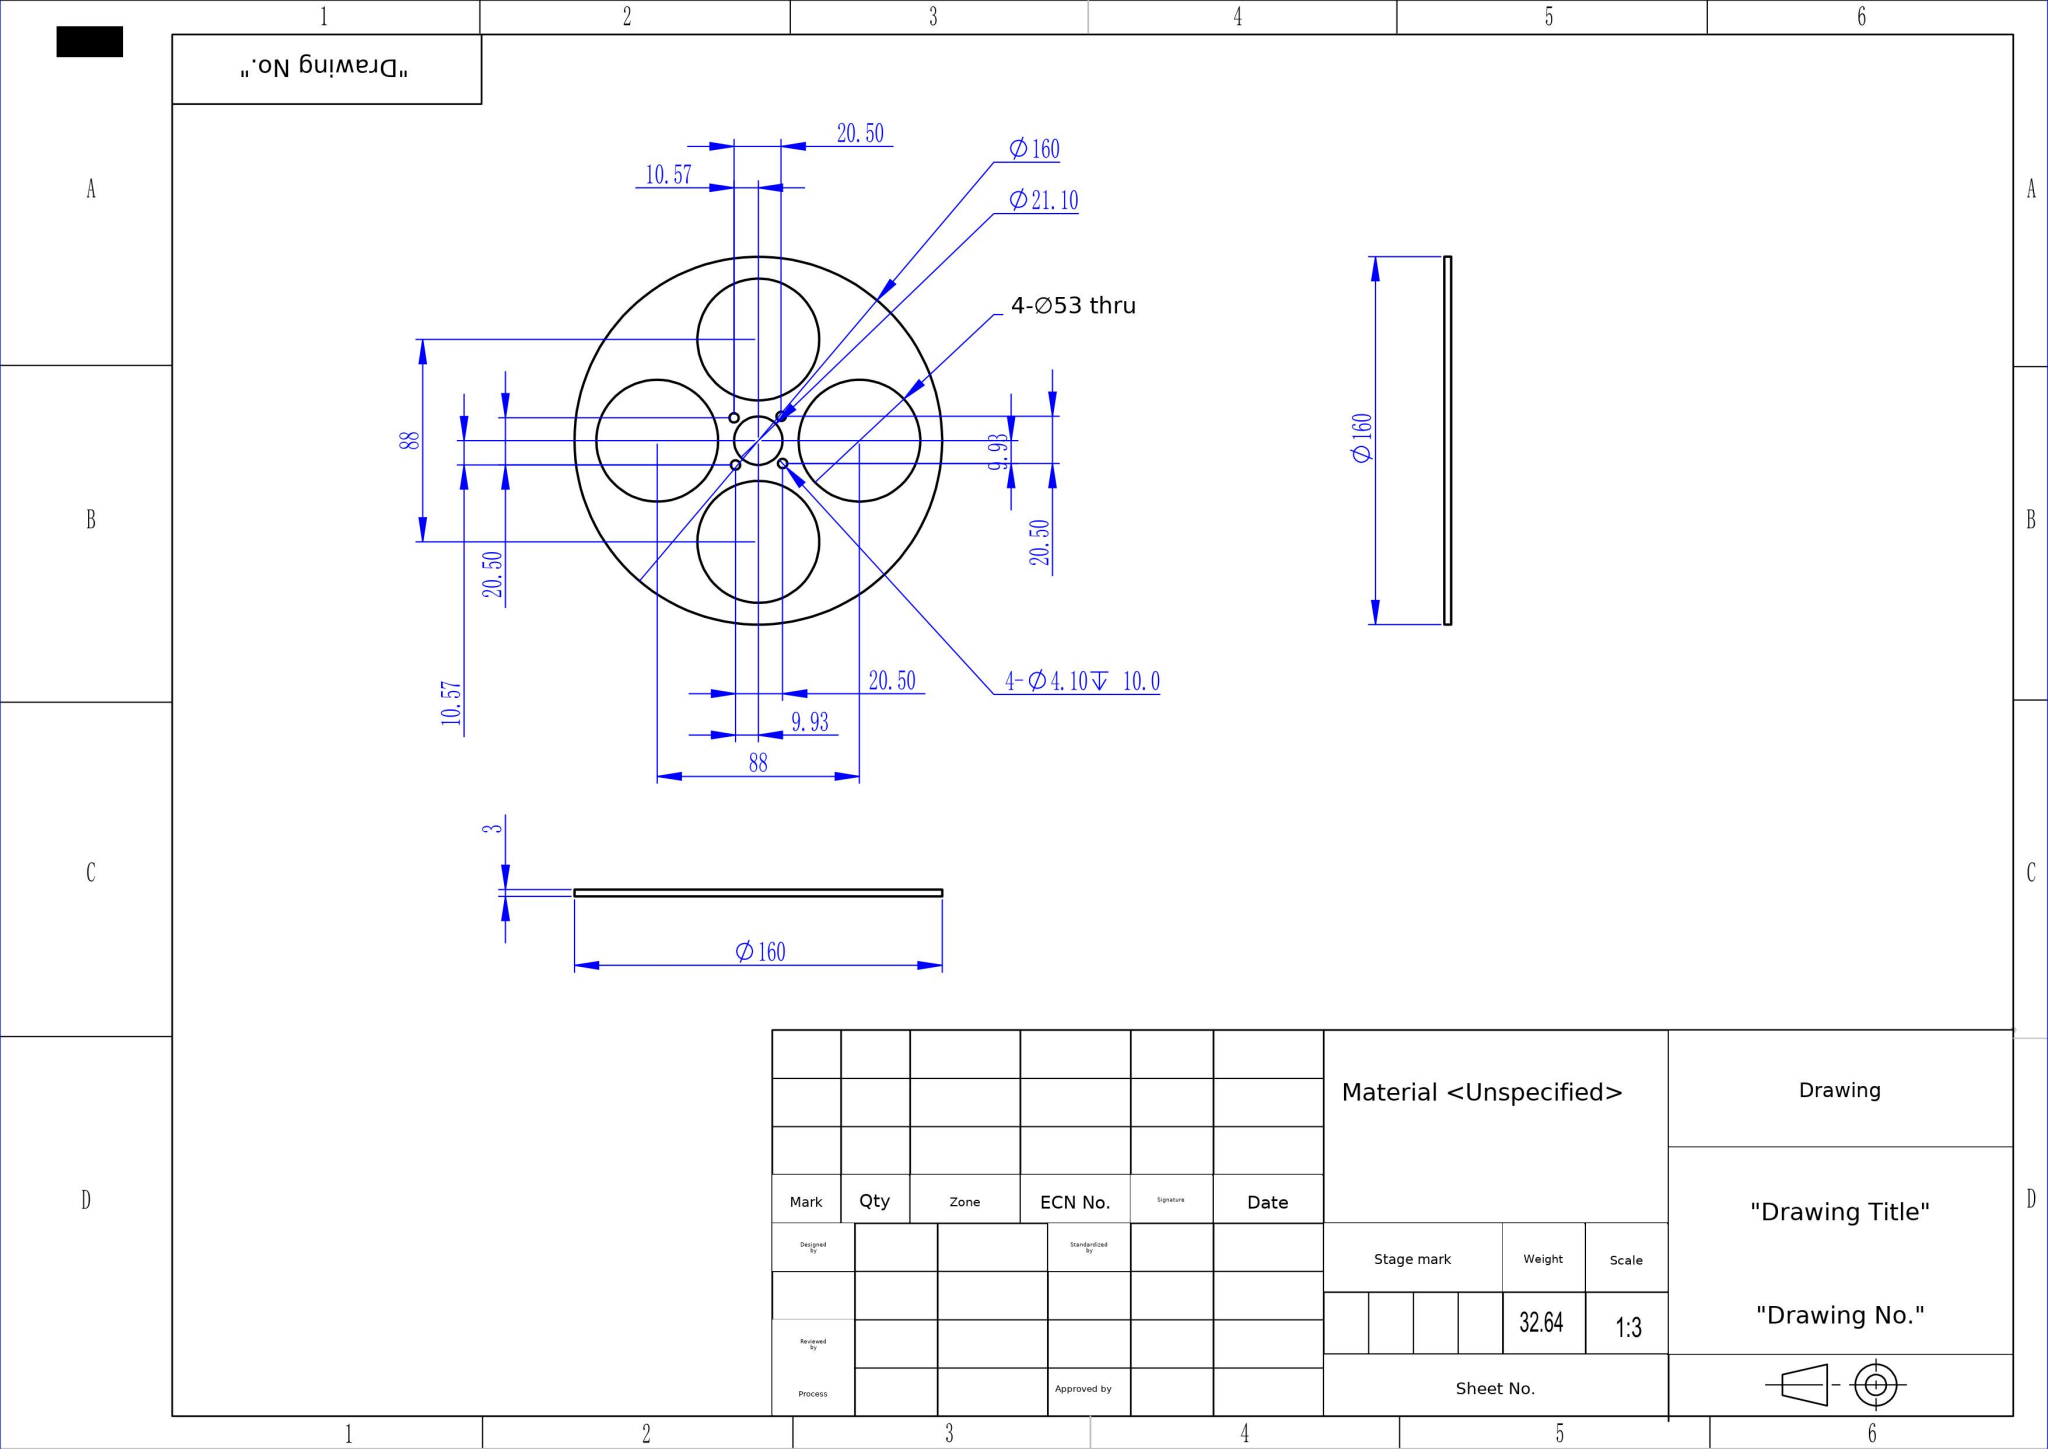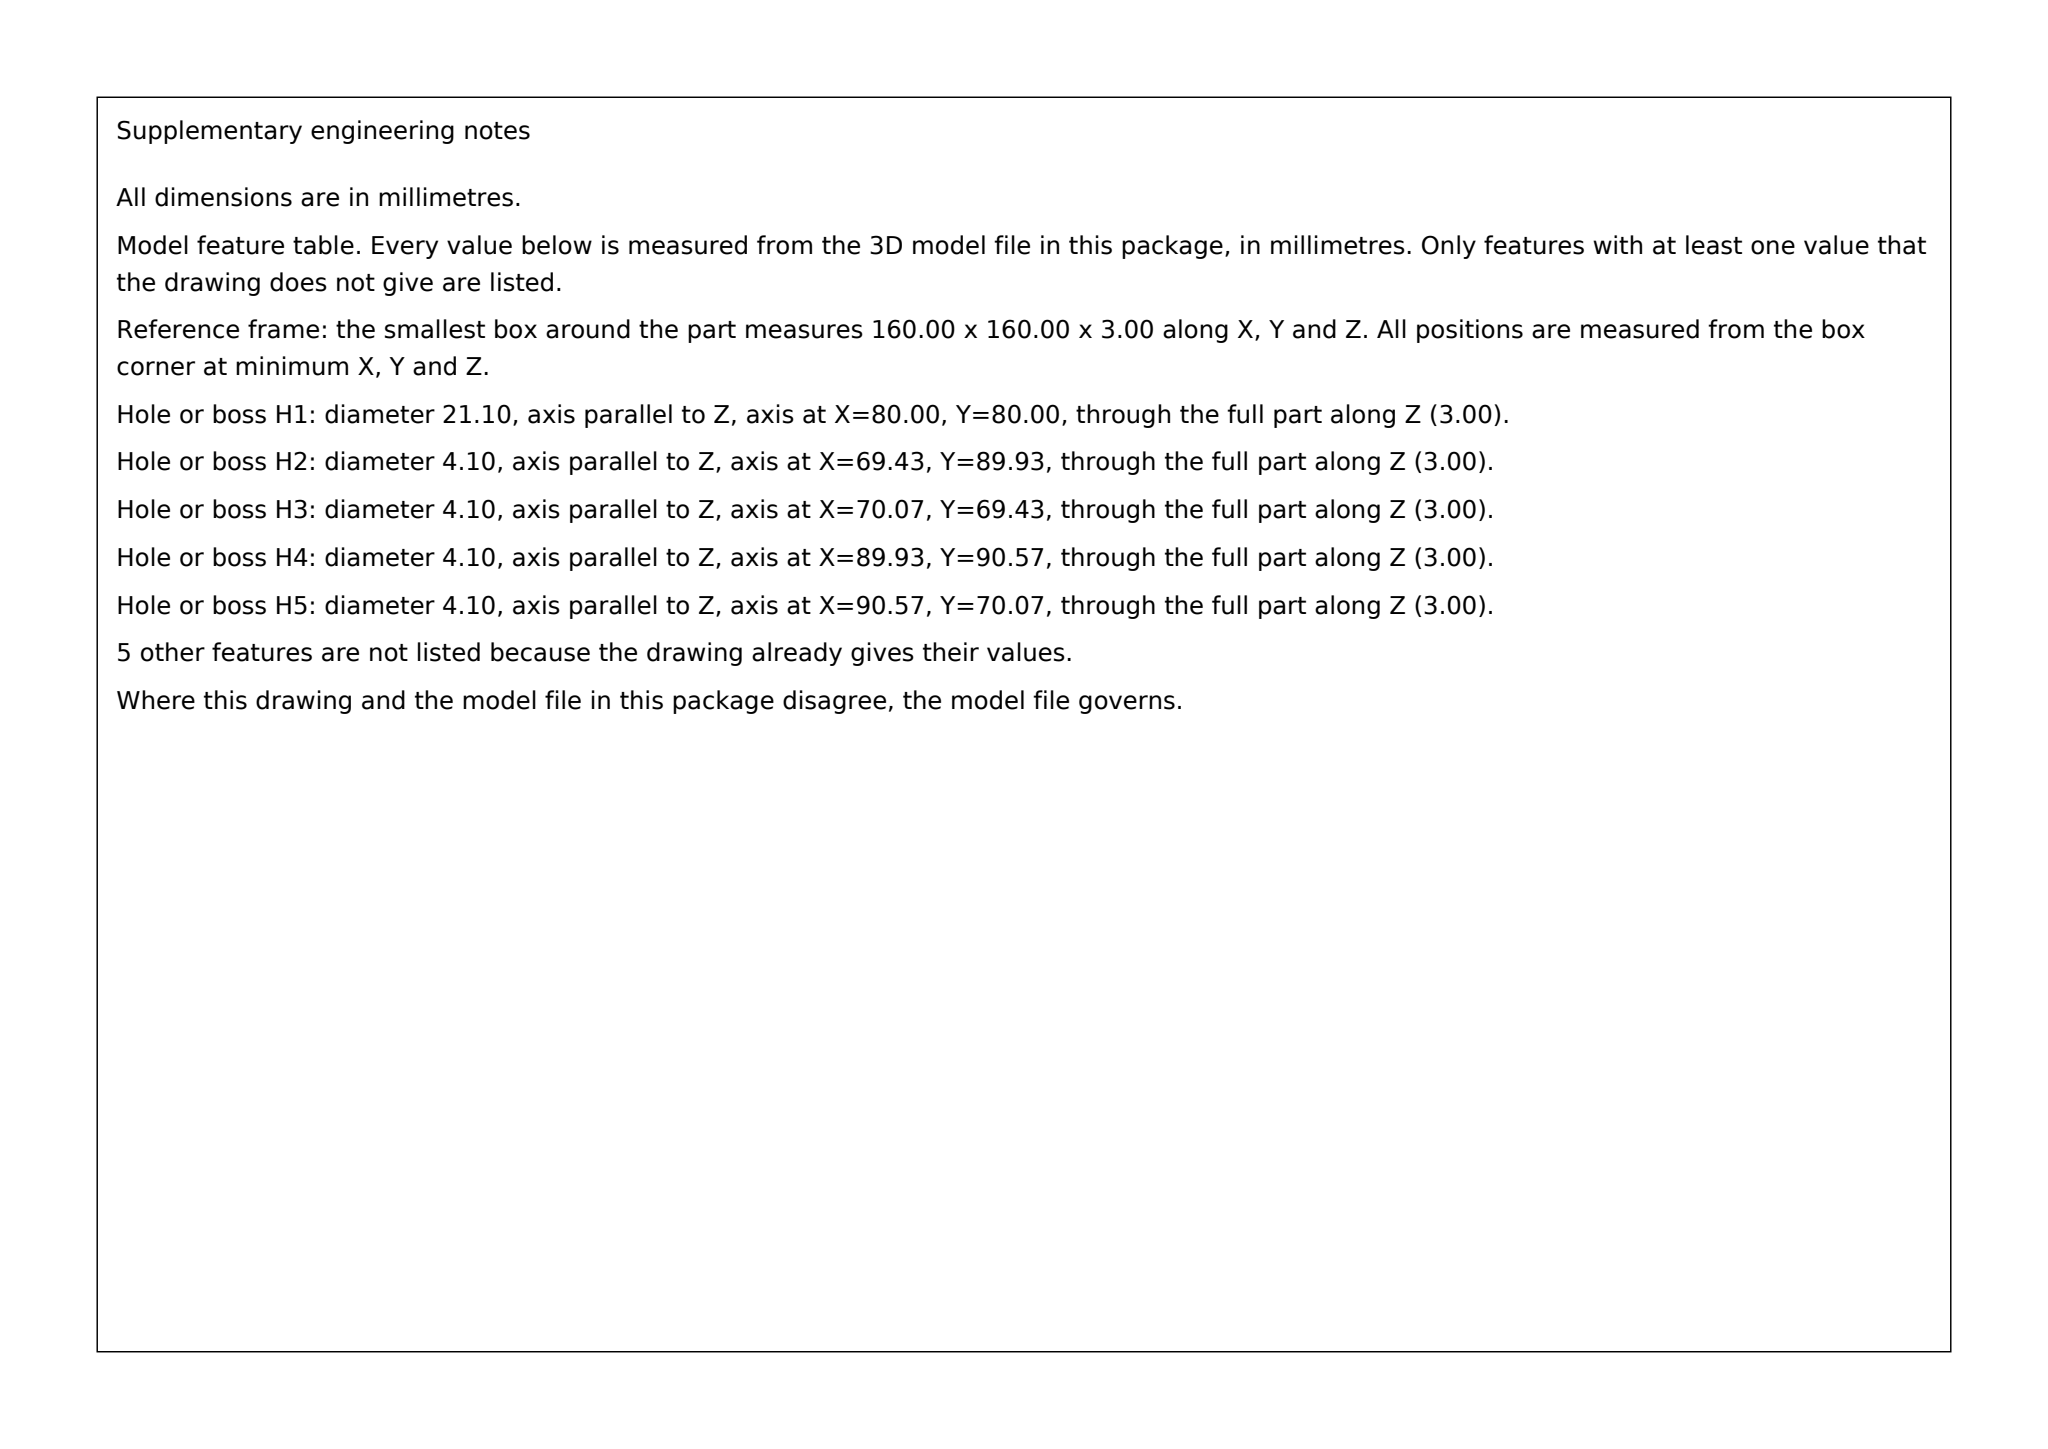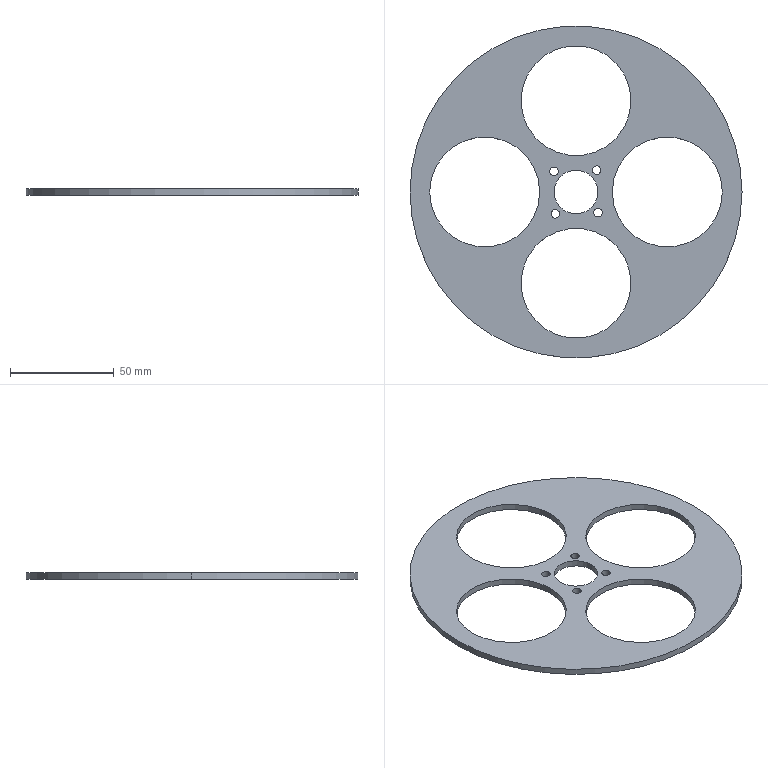Part | SolidWorks | mm | 1 solid | 22 faces | box 160 x 160 x 3 mm | volume 32637 mm3 | cylinder 20 | plane 2 | commonest cylinder face diameters 4.1 x8 53 x8 21.1 x2 160 x2
build123d program:
from build123d import *

# Parameters (mm, degrees)
SKETCH1_R           = 80
SKETCH1_R_2         = 10.55
BOSS_EXTRUDE1_DEPTH = 3
CUT_EXTRUDE1_REACH  = 115.177
SKETCH2_R           = 26.5
CIRPATTERN1_COUNT   = 4
SKETCH3_R           = 2.05
CUT_EXTRUDE2_DEPTH  = 10


with BuildPart() as part:
    # Sketch1 → Boss-Extrude1 (new body)
    with BuildSketch(Plane.XY):
        Circle(SKETCH1_R)
        Circle(SKETCH1_R_2, mode=Mode.SUBTRACT)
    extrude(amount=BOSS_EXTRUDE1_DEPTH)

    # Sketch2 → Cut-Extrude1 (cut, up to next)
    with BuildSketch(Plane.XY.offset(3), mode=Mode.PRIVATE) as cut_extrude1_sk1:
        with Locations((0, 44)):
            Circle(SKETCH2_R)
    cut_extrude1_tool1 = extrude(cut_extrude1_sk1.sketch, amount=-CUT_EXTRUDE1_REACH, mode=Mode.PRIVATE) & part.part
    cut_extrude1 = cut_extrude1_tool1.solids().sort_by_distance((0, 44, 3))[0]
    add(cut_extrude1, mode=Mode.SUBTRACT)

    # CirPattern1: Cut-Extrude1 ×4 about axis
    cirpattern1_axis = Axis((0, 0, 0), (0, 0, 1))
    for i in range(1, CIRPATTERN1_COUNT):
        add(cut_extrude1.rotate(cirpattern1_axis, i * 360 / CIRPATTERN1_COUNT), mode=Mode.SUBTRACT)

    # Sketch3 → Cut-Extrude2 (cut)
    with BuildSketch(Plane.XY.offset(3)):
        with Locations((9.929, 10.567)):
            Circle(SKETCH3_R)
        with Locations((10.567, -9.929)):
            Circle(SKETCH3_R)
        with Locations((-9.929, -10.567)):
            Circle(SKETCH3_R)
        with Locations((-10.567, 9.929)):
            Circle(SKETCH3_R)
    extrude(amount=-CUT_EXTRUDE2_DEPTH, mode=Mode.SUBTRACT)


solid = part.part
STEP:
#1=CARTESIAN_POINT('',(-12.617,9.929,0.));
#2=VERTEX_POINT('',#1);
#3=CARTESIAN_POINT('',(-8.517,9.929,0.));
#4=VERTEX_POINT('',#3);
#5=CARTESIAN_POINT('',(-10.567,9.929,0.));
#6=DIRECTION('',(0.,0.,1.));
#7=DIRECTION('',(1.,0.,0.));
#8=AXIS2_PLACEMENT_3D('',#5,#6,#7);
#9=CIRCLE('',#8,2.05);
#10=EDGE_CURVE('',#2,#4,#9,.T.);
#11=ORIENTED_EDGE('',*,*,#10,.F.);
#12=CARTESIAN_POINT('',(-12.617,9.929,3.));
#13=VERTEX_POINT('',#12);
#14=CARTESIAN_POINT('',(-12.617,9.929,-7.));
#15=DIRECTION('',(0.,0.,1.));
#16=VECTOR('',#15,1000.);
#17=LINE('',#14,#16);
#18=EDGE_CURVE('',#2,#13,#17,.T.);
#19=ORIENTED_EDGE('',*,*,#18,.T.);
#20=CARTESIAN_POINT('',(-8.517,9.929,3.));
#21=VERTEX_POINT('',#20);
#22=CARTESIAN_POINT('',(-10.567,9.929,3.));
#23=DIRECTION('',(0.,0.,1.));
#24=DIRECTION('',(1.,0.,0.));
#25=AXIS2_PLACEMENT_3D('',#22,#23,#24);
#26=CIRCLE('',#25,2.05);
#27=EDGE_CURVE('',#13,#21,#26,.T.);
#28=ORIENTED_EDGE('',*,*,#27,.T.);
#29=CARTESIAN_POINT('',(-8.517,9.929,-7.));
#30=DIRECTION('',(0.,0.,1.));
#31=VECTOR('',#30,1000.);
#32=LINE('',#29,#31);
#33=EDGE_CURVE('',#4,#21,#32,.T.);
#34=ORIENTED_EDGE('',*,*,#33,.F.);
#35=EDGE_LOOP('',(#11,#19,#28,#34));
#36=FACE_OUTER_BOUND('',#35,.T.);
#37=CARTESIAN_POINT('',(-10.567,9.929,-7.));
#38=DIRECTION('',(0.,0.,1.));
#39=DIRECTION('',(1.,0.,0.));
#40=AXIS2_PLACEMENT_3D('',#37,#38,#39);
#41=CYLINDRICAL_SURFACE('',#40,2.05);
#42=ADVANCED_FACE('',(#36),#41,.F.);
#43=CARTESIAN_POINT('',(-11.979,-10.567,0.));
#44=VERTEX_POINT('',#43);
#45=CARTESIAN_POINT('',(-7.879,-10.567,0.));
#46=VERTEX_POINT('',#45);
#47=CARTESIAN_POINT('',(-9.929,-10.567,0.));
#48=DIRECTION('',(0.,0.,1.));
#49=DIRECTION('',(1.,0.,0.));
#50=AXIS2_PLACEMENT_3D('',#47,#48,#49);
#51=CIRCLE('',#50,2.05);
#52=EDGE_CURVE('',#44,#46,#51,.T.);
#53=ORIENTED_EDGE('',*,*,#52,.F.);
#54=CARTESIAN_POINT('',(-11.979,-10.567,3.));
#55=VERTEX_POINT('',#54);
#56=CARTESIAN_POINT('',(-11.979,-10.567,-7.));
#57=DIRECTION('',(0.,0.,1.));
#58=VECTOR('',#57,1000.);
#59=LINE('',#56,#58);
#60=EDGE_CURVE('',#44,#55,#59,.T.);
#61=ORIENTED_EDGE('',*,*,#60,.T.);
#62=CARTESIAN_POINT('',(-7.879,-10.567,3.));
#63=VERTEX_POINT('',#62);
#64=CARTESIAN_POINT('',(-9.929,-10.567,3.));
#65=DIRECTION('',(0.,0.,1.));
#66=DIRECTION('',(1.,0.,0.));
#67=AXIS2_PLACEMENT_3D('',#64,#65,#66);
#68=CIRCLE('',#67,2.05);
#69=EDGE_CURVE('',#55,#63,#68,.T.);
#70=ORIENTED_EDGE('',*,*,#69,.T.);
#71=CARTESIAN_POINT('',(-7.879,-10.567,-7.));
#72=DIRECTION('',(0.,0.,1.));
#73=VECTOR('',#72,1000.);
#74=LINE('',#71,#73);
#75=EDGE_CURVE('',#46,#63,#74,.T.);
#76=ORIENTED_EDGE('',*,*,#75,.F.);
#77=EDGE_LOOP('',(#53,#61,#70,#76));
#78=FACE_OUTER_BOUND('',#77,.T.);
#79=CARTESIAN_POINT('',(-9.929,-10.567,-7.));
#80=DIRECTION('',(0.,0.,1.));
#81=DIRECTION('',(1.,0.,0.));
#82=AXIS2_PLACEMENT_3D('',#79,#80,#81);
#83=CYLINDRICAL_SURFACE('',#82,2.05);
#84=ADVANCED_FACE('',(#78),#83,.F.);
#85=CARTESIAN_POINT('',(8.517,-9.929,0.));
#86=VERTEX_POINT('',#85);
#87=CARTESIAN_POINT('',(12.617,-9.929,0.));
#88=VERTEX_POINT('',#87);
#89=CARTESIAN_POINT('',(10.567,-9.929,0.));
#90=DIRECTION('',(0.,0.,1.));
#91=DIRECTION('',(1.,0.,0.));
#92=AXIS2_PLACEMENT_3D('',#89,#90,#91);
#93=CIRCLE('',#92,2.05);
#94=EDGE_CURVE('',#86,#88,#93,.T.);
#95=ORIENTED_EDGE('',*,*,#94,.F.);
#96=CARTESIAN_POINT('',(8.517,-9.929,3.));
#97=VERTEX_POINT('',#96);
#98=CARTESIAN_POINT('',(8.517,-9.929,-7.));
#99=DIRECTION('',(0.,0.,1.));
#100=VECTOR('',#99,1000.);
#101=LINE('',#98,#100);
#102=EDGE_CURVE('',#86,#97,#101,.T.);
#103=ORIENTED_EDGE('',*,*,#102,.T.);
#104=CARTESIAN_POINT('',(12.617,-9.929,3.));
#105=VERTEX_POINT('',#104);
#106=CARTESIAN_POINT('',(10.567,-9.929,3.));
#107=DIRECTION('',(0.,0.,1.));
#108=DIRECTION('',(1.,0.,0.));
#109=AXIS2_PLACEMENT_3D('',#106,#107,#108);
#110=CIRCLE('',#109,2.05);
#111=EDGE_CURVE('',#97,#105,#110,.T.);
#112=ORIENTED_EDGE('',*,*,#111,.T.);
#113=CARTESIAN_POINT('',(12.617,-9.929,-7.));
#114=DIRECTION('',(0.,0.,1.));
#115=VECTOR('',#114,1000.);
#116=LINE('',#113,#115);
#117=EDGE_CURVE('',#88,#105,#116,.T.);
#118=ORIENTED_EDGE('',*,*,#117,.F.);
#119=EDGE_LOOP('',(#95,#103,#112,#118));
#120=FACE_OUTER_BOUND('',#119,.T.);
#121=CARTESIAN_POINT('',(10.567,-9.929,-7.));
#122=DIRECTION('',(0.,0.,1.));
#123=DIRECTION('',(1.,0.,0.));
#124=AXIS2_PLACEMENT_3D('',#121,#122,#123);
#125=CYLINDRICAL_SURFACE('',#124,2.05);
#126=ADVANCED_FACE('',(#120),#125,.F.);
#127=CARTESIAN_POINT('',(7.879,10.567,0.));
#128=VERTEX_POINT('',#127);
#129=CARTESIAN_POINT('',(11.979,10.567,0.));
#130=VERTEX_POINT('',#129);
#131=CARTESIAN_POINT('',(9.929,10.567,0.));
#132=DIRECTION('',(0.,0.,1.));
#133=DIRECTION('',(1.,0.,0.));
#134=AXIS2_PLACEMENT_3D('',#131,#132,#133);
#135=CIRCLE('',#134,2.05);
#136=EDGE_CURVE('',#128,#130,#135,.T.);
#137=ORIENTED_EDGE('',*,*,#136,.F.);
#138=CARTESIAN_POINT('',(7.879,10.567,3.));
#139=VERTEX_POINT('',#138);
#140=CARTESIAN_POINT('',(7.879,10.567,-7.));
#141=DIRECTION('',(0.,0.,1.));
#142=VECTOR('',#141,1000.);
#143=LINE('',#140,#142);
#144=EDGE_CURVE('',#128,#139,#143,.T.);
#145=ORIENTED_EDGE('',*,*,#144,.T.);
#146=CARTESIAN_POINT('',(11.979,10.567,3.));
#147=VERTEX_POINT('',#146);
#148=CARTESIAN_POINT('',(9.929,10.567,3.));
#149=DIRECTION('',(0.,0.,1.));
#150=DIRECTION('',(1.,0.,0.));
#151=AXIS2_PLACEMENT_3D('',#148,#149,#150);
#152=CIRCLE('',#151,2.05);
#153=EDGE_CURVE('',#139,#147,#152,.T.);
#154=ORIENTED_EDGE('',*,*,#153,.T.);
#155=CARTESIAN_POINT('',(11.979,10.567,-7.));
#156=DIRECTION('',(0.,0.,1.));
#157=VECTOR('',#156,1000.);
#158=LINE('',#155,#157);
#159=EDGE_CURVE('',#130,#147,#158,.T.);
#160=ORIENTED_EDGE('',*,*,#159,.F.);
#161=EDGE_LOOP('',(#137,#145,#154,#160));
#162=FACE_OUTER_BOUND('',#161,.T.);
#163=CARTESIAN_POINT('',(9.929,10.567,-7.));
#164=DIRECTION('',(0.,0.,1.));
#165=DIRECTION('',(1.,0.,0.));
#166=AXIS2_PLACEMENT_3D('',#163,#164,#165);
#167=CYLINDRICAL_SURFACE('',#166,2.05);
#168=ADVANCED_FACE('',(#162),#167,.F.);
#169=CARTESIAN_POINT('',(26.5,-44.,0.));
#170=VERTEX_POINT('',#169);
#171=CARTESIAN_POINT('',(-26.5,-44.,0.));
#172=VERTEX_POINT('',#171);
#173=CARTESIAN_POINT('',(0.,-44.,0.));
#174=DIRECTION('',(0.,0.,-1.));
#175=DIRECTION('',(1.,0.,0.));
#176=AXIS2_PLACEMENT_3D('',#173,#174,#175);
#177=CIRCLE('',#176,26.5);
#178=EDGE_CURVE('',#170,#172,#177,.T.);
#179=ORIENTED_EDGE('',*,*,#178,.T.);
#180=CARTESIAN_POINT('',(-26.5,-44.,3.));
#181=VERTEX_POINT('',#180);
#182=CARTESIAN_POINT('',(-26.5,-44.,-0.001));
#183=DIRECTION('',(0.,0.,1.));
#184=VECTOR('',#183,1000.);
#185=LINE('',#182,#184);
#186=EDGE_CURVE('',#172,#181,#185,.T.);
#187=ORIENTED_EDGE('',*,*,#186,.T.);
#188=CARTESIAN_POINT('',(26.5,-44.,3.));
#189=VERTEX_POINT('',#188);
#190=CARTESIAN_POINT('',(0.,-44.,3.));
#191=DIRECTION('',(0.,0.,1.));
#192=DIRECTION('',(-1.,0.,0.));
#193=AXIS2_PLACEMENT_3D('',#190,#191,#192);
#194=CIRCLE('',#193,26.5);
#195=EDGE_CURVE('',#181,#189,#194,.T.);
#196=ORIENTED_EDGE('',*,*,#195,.T.);
#197=CARTESIAN_POINT('',(26.5,-44.,-0.001));
#198=DIRECTION('',(0.,0.,1.));
#199=VECTOR('',#198,1000.);
#200=LINE('',#197,#199);
#201=EDGE_CURVE('',#170,#189,#200,.T.);
#202=ORIENTED_EDGE('',*,*,#201,.F.);
#203=EDGE_LOOP('',(#179,#187,#196,#202));
#204=FACE_OUTER_BOUND('',#203,.T.);
#205=CARTESIAN_POINT('',(0.,-44.,-0.001));
#206=DIRECTION('',(0.,0.,1.));
#207=DIRECTION('',(1.,0.,0.));
#208=AXIS2_PLACEMENT_3D('',#205,#206,#207);
#209=CYLINDRICAL_SURFACE('',#208,26.5);
#210=ADVANCED_FACE('',(#204),#209,.F.);
#211=CARTESIAN_POINT('',(-17.5,0.,0.));
#212=VERTEX_POINT('',#211);
#213=CARTESIAN_POINT('',(-70.5,0.,0.));
#214=VERTEX_POINT('',#213);
#215=CARTESIAN_POINT('',(-44.,0.,0.));
#216=DIRECTION('',(0.,0.,-1.));
#217=DIRECTION('',(1.,0.,0.));
#218=AXIS2_PLACEMENT_3D('',#215,#216,#217);
#219=CIRCLE('',#218,26.5);
#220=EDGE_CURVE('',#212,#214,#219,.T.);
#221=ORIENTED_EDGE('',*,*,#220,.T.);
#222=CARTESIAN_POINT('',(-70.5,0.,3.));
#223=VERTEX_POINT('',#222);
#224=CARTESIAN_POINT('',(-70.5,0.,-0.001));
#225=DIRECTION('',(0.,0.,1.));
#226=VECTOR('',#225,1000.);
#227=LINE('',#224,#226);
#228=EDGE_CURVE('',#214,#223,#227,.T.);
#229=ORIENTED_EDGE('',*,*,#228,.T.);
#230=CARTESIAN_POINT('',(-17.5,0.,3.));
#231=VERTEX_POINT('',#230);
#232=CARTESIAN_POINT('',(-44.,0.,3.));
#233=DIRECTION('',(0.,0.,1.));
#234=DIRECTION('',(0.,1.,0.));
#235=AXIS2_PLACEMENT_3D('',#232,#233,#234);
#236=CIRCLE('',#235,26.5);
#237=EDGE_CURVE('',#223,#231,#236,.T.);
#238=ORIENTED_EDGE('',*,*,#237,.T.);
#239=CARTESIAN_POINT('',(-17.5,0.,-0.001));
#240=DIRECTION('',(0.,0.,1.));
#241=VECTOR('',#240,1000.);
#242=LINE('',#239,#241);
#243=EDGE_CURVE('',#212,#231,#242,.T.);
#244=ORIENTED_EDGE('',*,*,#243,.F.);
#245=EDGE_LOOP('',(#221,#229,#238,#244));
#246=FACE_OUTER_BOUND('',#245,.T.);
#247=CARTESIAN_POINT('',(-44.,0.,-0.001));
#248=DIRECTION('',(0.,0.,1.));
#249=DIRECTION('',(1.,0.,0.));
#250=AXIS2_PLACEMENT_3D('',#247,#248,#249);
#251=CYLINDRICAL_SURFACE('',#250,26.5);
#252=ADVANCED_FACE('',(#246),#251,.F.);
#253=CARTESIAN_POINT('',(70.5,-0.,0.));
#254=VERTEX_POINT('',#253);
#255=CARTESIAN_POINT('',(17.5,-0.,0.));
#256=VERTEX_POINT('',#255);
#257=CARTESIAN_POINT('',(44.,-0.,0.));
#258=DIRECTION('',(0.,0.,-1.));
#259=DIRECTION('',(1.,0.,0.));
#260=AXIS2_PLACEMENT_3D('',#257,#258,#259);
#261=CIRCLE('',#260,26.5);
#262=EDGE_CURVE('',#254,#256,#261,.T.);
#263=ORIENTED_EDGE('',*,*,#262,.T.);
#264=CARTESIAN_POINT('',(17.5,-0.,3.));
#265=VERTEX_POINT('',#264);
#266=CARTESIAN_POINT('',(17.5,-0.,-0.001));
#267=DIRECTION('',(0.,0.,1.));
#268=VECTOR('',#267,1000.);
#269=LINE('',#266,#268);
#270=EDGE_CURVE('',#256,#265,#269,.T.);
#271=ORIENTED_EDGE('',*,*,#270,.T.);
#272=CARTESIAN_POINT('',(70.5,-0.,3.));
#273=VERTEX_POINT('',#272);
#274=CARTESIAN_POINT('',(44.,-0.,3.));
#275=DIRECTION('',(0.,0.,1.));
#276=DIRECTION('',(-0.,-1.,0.));
#277=AXIS2_PLACEMENT_3D('',#274,#275,#276);
#278=CIRCLE('',#277,26.5);
#279=EDGE_CURVE('',#265,#273,#278,.T.);
#280=ORIENTED_EDGE('',*,*,#279,.T.);
#281=CARTESIAN_POINT('',(70.5,-0.,-0.001));
#282=DIRECTION('',(0.,0.,1.));
#283=VECTOR('',#282,1000.);
#284=LINE('',#281,#283);
#285=EDGE_CURVE('',#254,#273,#284,.T.);
#286=ORIENTED_EDGE('',*,*,#285,.F.);
#287=EDGE_LOOP('',(#263,#271,#280,#286));
#288=FACE_OUTER_BOUND('',#287,.T.);
#289=CARTESIAN_POINT('',(44.,-0.,-0.001));
#290=DIRECTION('',(0.,0.,1.));
#291=DIRECTION('',(1.,0.,0.));
#292=AXIS2_PLACEMENT_3D('',#289,#290,#291);
#293=CYLINDRICAL_SURFACE('',#292,26.5);
#294=ADVANCED_FACE('',(#288),#293,.F.);
#295=CARTESIAN_POINT('',(26.5,44.,0.));
#296=VERTEX_POINT('',#295);
#297=CARTESIAN_POINT('',(-26.5,44.,0.));
#298=VERTEX_POINT('',#297);
#299=CARTESIAN_POINT('',(0.,44.,0.));
#300=DIRECTION('',(0.,0.,-1.));
#301=DIRECTION('',(1.,0.,0.));
#302=AXIS2_PLACEMENT_3D('',#299,#300,#301);
#303=CIRCLE('',#302,26.5);
#304=EDGE_CURVE('',#296,#298,#303,.T.);
#305=ORIENTED_EDGE('',*,*,#304,.T.);
#306=CARTESIAN_POINT('',(-26.5,44.,3.));
#307=VERTEX_POINT('',#306);
#308=CARTESIAN_POINT('',(-26.5,44.,-0.001));
#309=DIRECTION('',(0.,0.,1.));
#310=VECTOR('',#309,1000.);
#311=LINE('',#308,#310);
#312=EDGE_CURVE('',#298,#307,#311,.T.);
#313=ORIENTED_EDGE('',*,*,#312,.T.);
#314=CARTESIAN_POINT('',(26.5,44.,3.));
#315=VERTEX_POINT('',#314);
#316=CARTESIAN_POINT('',(0.,44.,3.));
#317=DIRECTION('',(0.,0.,1.));
#318=DIRECTION('',(1.,0.,0.));
#319=AXIS2_PLACEMENT_3D('',#316,#317,#318);
#320=CIRCLE('',#319,26.5);
#321=EDGE_CURVE('',#307,#315,#320,.T.);
#322=ORIENTED_EDGE('',*,*,#321,.T.);
#323=CARTESIAN_POINT('',(26.5,44.,-0.001));
#324=DIRECTION('',(0.,0.,1.));
#325=VECTOR('',#324,1000.);
#326=LINE('',#323,#325);
#327=EDGE_CURVE('',#296,#315,#326,.T.);
#328=ORIENTED_EDGE('',*,*,#327,.F.);
#329=EDGE_LOOP('',(#305,#313,#322,#328));
#330=FACE_OUTER_BOUND('',#329,.T.);
#331=CARTESIAN_POINT('',(0.,44.,-0.001));
#332=DIRECTION('',(0.,0.,1.));
#333=DIRECTION('',(1.,0.,0.));
#334=AXIS2_PLACEMENT_3D('',#331,#332,#333);
#335=CYLINDRICAL_SURFACE('',#334,26.5);
#336=ADVANCED_FACE('',(#330),#335,.F.);
#337=CARTESIAN_POINT('',(-10.55,0.,3.));
#338=VERTEX_POINT('',#337);
#339=CARTESIAN_POINT('',(10.55,0.,3.));
#340=VERTEX_POINT('',#339);
#341=CARTESIAN_POINT('',(0.,0.,3.));
#342=DIRECTION('',(0.,0.,1.));
#343=DIRECTION('',(1.,0.,0.));
#344=AXIS2_PLACEMENT_3D('',#341,#342,#343);
#345=CIRCLE('',#344,10.55);
#346=EDGE_CURVE('',#338,#340,#345,.T.);
#347=ORIENTED_EDGE('',*,*,#346,.T.);
#348=CARTESIAN_POINT('',(10.55,0.,0.));
#349=VERTEX_POINT('',#348);
#350=CARTESIAN_POINT('',(10.55,0.,3.));
#351=DIRECTION('',(0.,0.,-1.));
#352=VECTOR('',#351,1000.);
#353=LINE('',#350,#352);
#354=EDGE_CURVE('',#340,#349,#353,.T.);
#355=ORIENTED_EDGE('',*,*,#354,.T.);
#356=CARTESIAN_POINT('',(-10.55,0.,0.));
#357=VERTEX_POINT('',#356);
#358=CARTESIAN_POINT('',(0.,0.,0.));
#359=DIRECTION('',(0.,0.,1.));
#360=DIRECTION('',(1.,0.,0.));
#361=AXIS2_PLACEMENT_3D('',#358,#359,#360);
#362=CIRCLE('',#361,10.55);
#363=EDGE_CURVE('',#357,#349,#362,.T.);
#364=ORIENTED_EDGE('',*,*,#363,.F.);
#365=CARTESIAN_POINT('',(-10.55,0.,3.));
#366=DIRECTION('',(0.,0.,-1.));
#367=VECTOR('',#366,1000.);
#368=LINE('',#365,#367);
#369=EDGE_CURVE('',#338,#357,#368,.T.);
#370=ORIENTED_EDGE('',*,*,#369,.F.);
#371=EDGE_LOOP('',(#347,#355,#364,#370));
#372=FACE_OUTER_BOUND('',#371,.T.);
#373=CARTESIAN_POINT('',(0.,0.,3.));
#374=DIRECTION('',(0.,0.,-1.));
#375=DIRECTION('',(-1.,0.,0.));
#376=AXIS2_PLACEMENT_3D('',#373,#374,#375);
#377=CYLINDRICAL_SURFACE('',#376,10.55);
#378=ADVANCED_FACE('',(#372),#377,.F.);
#379=CARTESIAN_POINT('',(80.,0.,3.));
#380=VERTEX_POINT('',#379);
#381=CARTESIAN_POINT('',(-80.,0.,3.));
#382=VERTEX_POINT('',#381);
#383=CARTESIAN_POINT('',(0.,0.,3.));
#384=DIRECTION('',(0.,0.,1.));
#385=DIRECTION('',(1.,0.,0.));
#386=AXIS2_PLACEMENT_3D('',#383,#384,#385);
#387=CIRCLE('',#386,80.);
#388=EDGE_CURVE('',#380,#382,#387,.T.);
#389=ORIENTED_EDGE('',*,*,#388,.F.);
#390=CARTESIAN_POINT('',(80.,0.,0.));
#391=VERTEX_POINT('',#390);
#392=CARTESIAN_POINT('',(80.,0.,3.));
#393=DIRECTION('',(0.,0.,-1.));
#394=VECTOR('',#393,1000.);
#395=LINE('',#392,#394);
#396=EDGE_CURVE('',#380,#391,#395,.T.);
#397=ORIENTED_EDGE('',*,*,#396,.T.);
#398=CARTESIAN_POINT('',(-80.,0.,0.));
#399=VERTEX_POINT('',#398);
#400=CARTESIAN_POINT('',(0.,0.,0.));
#401=DIRECTION('',(0.,0.,1.));
#402=DIRECTION('',(1.,0.,0.));
#403=AXIS2_PLACEMENT_3D('',#400,#401,#402);
#404=CIRCLE('',#403,80.);
#405=EDGE_CURVE('',#391,#399,#404,.T.);
#406=ORIENTED_EDGE('',*,*,#405,.T.);
#407=CARTESIAN_POINT('',(-80.,0.,3.));
#408=DIRECTION('',(0.,0.,-1.));
#409=VECTOR('',#408,1000.);
#410=LINE('',#407,#409);
#411=EDGE_CURVE('',#382,#399,#410,.T.);
#412=ORIENTED_EDGE('',*,*,#411,.F.);
#413=EDGE_LOOP('',(#389,#397,#406,#412));
#414=FACE_OUTER_BOUND('',#413,.T.);
#415=CARTESIAN_POINT('',(0.,0.,3.));
#416=DIRECTION('',(0.,0.,-1.));
#417=DIRECTION('',(-1.,0.,0.));
#418=AXIS2_PLACEMENT_3D('',#415,#416,#417);
#419=CYLINDRICAL_SURFACE('',#418,80.);
#420=ADVANCED_FACE('',(#414),#419,.T.);
#421=CARTESIAN_POINT('',(-10.567,9.929,3.));
#422=DIRECTION('',(0.,0.,1.));
#423=DIRECTION('',(1.,0.,0.));
#424=AXIS2_PLACEMENT_3D('',#421,#422,#423);
#425=CIRCLE('',#424,2.05);
#426=EDGE_CURVE('',#21,#13,#425,.T.);
#427=ORIENTED_EDGE('',*,*,#426,.F.);
#428=ORIENTED_EDGE('',*,*,#27,.F.);
#429=EDGE_LOOP('',(#427,#428));
#430=FACE_BOUND('',#429,.T.);
#431=CARTESIAN_POINT('',(-9.929,-10.567,3.));
#432=DIRECTION('',(0.,0.,1.));
#433=DIRECTION('',(1.,0.,0.));
#434=AXIS2_PLACEMENT_3D('',#431,#432,#433);
#435=CIRCLE('',#434,2.05);
#436=EDGE_CURVE('',#63,#55,#435,.T.);
#437=ORIENTED_EDGE('',*,*,#436,.F.);
#438=ORIENTED_EDGE('',*,*,#69,.F.);
#439=EDGE_LOOP('',(#437,#438));
#440=FACE_BOUND('',#439,.T.);
#441=CARTESIAN_POINT('',(10.567,-9.929,3.));
#442=DIRECTION('',(0.,0.,1.));
#443=DIRECTION('',(1.,0.,0.));
#444=AXIS2_PLACEMENT_3D('',#441,#442,#443);
#445=CIRCLE('',#444,2.05);
#446=EDGE_CURVE('',#105,#97,#445,.T.);
#447=ORIENTED_EDGE('',*,*,#446,.F.);
#448=ORIENTED_EDGE('',*,*,#111,.F.);
#449=EDGE_LOOP('',(#447,#448));
#450=FACE_BOUND('',#449,.T.);
#451=CARTESIAN_POINT('',(9.929,10.567,3.));
#452=DIRECTION('',(0.,0.,1.));
#453=DIRECTION('',(1.,0.,0.));
#454=AXIS2_PLACEMENT_3D('',#451,#452,#453);
#455=CIRCLE('',#454,2.05);
#456=EDGE_CURVE('',#147,#139,#455,.T.);
#457=ORIENTED_EDGE('',*,*,#456,.F.);
#458=ORIENTED_EDGE('',*,*,#153,.F.);
#459=EDGE_LOOP('',(#457,#458));
#460=FACE_BOUND('',#459,.T.);
#461=CARTESIAN_POINT('',(0.,-44.,3.));
#462=DIRECTION('',(0.,0.,1.));
#463=DIRECTION('',(-1.,0.,0.));
#464=AXIS2_PLACEMENT_3D('',#461,#462,#463);
#465=CIRCLE('',#464,26.5);
#466=EDGE_CURVE('',#189,#181,#465,.T.);
#467=ORIENTED_EDGE('',*,*,#466,.F.);
#468=ORIENTED_EDGE('',*,*,#195,.F.);
#469=EDGE_LOOP('',(#467,#468));
#470=FACE_BOUND('',#469,.T.);
#471=CARTESIAN_POINT('',(-44.,0.,3.));
#472=DIRECTION('',(0.,0.,1.));
#473=DIRECTION('',(0.,1.,0.));
#474=AXIS2_PLACEMENT_3D('',#471,#472,#473);
#475=CIRCLE('',#474,26.5);
#476=EDGE_CURVE('',#231,#223,#475,.T.);
#477=ORIENTED_EDGE('',*,*,#476,.F.);
#478=ORIENTED_EDGE('',*,*,#237,.F.);
#479=EDGE_LOOP('',(#477,#478));
#480=FACE_BOUND('',#479,.T.);
#481=CARTESIAN_POINT('',(44.,-0.,3.));
#482=DIRECTION('',(0.,0.,1.));
#483=DIRECTION('',(-0.,-1.,0.));
#484=AXIS2_PLACEMENT_3D('',#481,#482,#483);
#485=CIRCLE('',#484,26.5);
#486=EDGE_CURVE('',#273,#265,#485,.T.);
#487=ORIENTED_EDGE('',*,*,#486,.F.);
#488=ORIENTED_EDGE('',*,*,#279,.F.);
#489=EDGE_LOOP('',(#487,#488));
#490=FACE_BOUND('',#489,.T.);
#491=CARTESIAN_POINT('',(0.,44.,3.));
#492=DIRECTION('',(0.,0.,1.));
#493=DIRECTION('',(1.,0.,0.));
#494=AXIS2_PLACEMENT_3D('',#491,#492,#493);
#495=CIRCLE('',#494,26.5);
#496=EDGE_CURVE('',#315,#307,#495,.T.);
#497=ORIENTED_EDGE('',*,*,#496,.F.);
#498=ORIENTED_EDGE('',*,*,#321,.F.);
#499=EDGE_LOOP('',(#497,#498));
#500=FACE_BOUND('',#499,.T.);
#501=CARTESIAN_POINT('',(0.,0.,3.));
#502=DIRECTION('',(0.,0.,1.));
#503=DIRECTION('',(1.,0.,0.));
#504=AXIS2_PLACEMENT_3D('',#501,#502,#503);
#505=CIRCLE('',#504,80.);
#506=EDGE_CURVE('',#382,#380,#505,.T.);
#507=ORIENTED_EDGE('',*,*,#506,.T.);
#508=ORIENTED_EDGE('',*,*,#388,.T.);
#509=EDGE_LOOP('',(#507,#508));
#510=FACE_OUTER_BOUND('',#509,.T.);
#511=ORIENTED_EDGE('',*,*,#346,.F.);
#512=CARTESIAN_POINT('',(0.,0.,3.));
#513=DIRECTION('',(0.,0.,1.));
#514=DIRECTION('',(1.,0.,0.));
#515=AXIS2_PLACEMENT_3D('',#512,#513,#514);
#516=CIRCLE('',#515,10.55);
#517=EDGE_CURVE('',#340,#338,#516,.T.);
#518=ORIENTED_EDGE('',*,*,#517,.F.);
#519=EDGE_LOOP('',(#511,#518));
#520=FACE_BOUND('',#519,.T.);
#521=CARTESIAN_POINT('',(0.,0.,3.));
#522=DIRECTION('',(0.,0.,1.));
#523=DIRECTION('',(1.,0.,0.));
#524=AXIS2_PLACEMENT_3D('',#521,#522,#523);
#525=PLANE('',#524);
#526=ADVANCED_FACE('',(#430,#440,#450,#460,#470,#480,#490,#500,#510,#520),#525,.T.);
#527=CARTESIAN_POINT('',(-10.567,9.929,0.));
#528=DIRECTION('',(0.,0.,1.));
#529=DIRECTION('',(1.,0.,0.));
#530=AXIS2_PLACEMENT_3D('',#527,#528,#529);
#531=CIRCLE('',#530,2.05);
#532=EDGE_CURVE('',#4,#2,#531,.T.);
#533=ORIENTED_EDGE('',*,*,#532,.T.);
#534=ORIENTED_EDGE('',*,*,#10,.T.);
#535=EDGE_LOOP('',(#533,#534));
#536=FACE_BOUND('',#535,.T.);
#537=CARTESIAN_POINT('',(-9.929,-10.567,0.));
#538=DIRECTION('',(0.,0.,1.));
#539=DIRECTION('',(1.,0.,0.));
#540=AXIS2_PLACEMENT_3D('',#537,#538,#539);
#541=CIRCLE('',#540,2.05);
#542=EDGE_CURVE('',#46,#44,#541,.T.);
#543=ORIENTED_EDGE('',*,*,#542,.T.);
#544=ORIENTED_EDGE('',*,*,#52,.T.);
#545=EDGE_LOOP('',(#543,#544));
#546=FACE_BOUND('',#545,.T.);
#547=CARTESIAN_POINT('',(10.567,-9.929,0.));
#548=DIRECTION('',(0.,0.,1.));
#549=DIRECTION('',(1.,0.,0.));
#550=AXIS2_PLACEMENT_3D('',#547,#548,#549);
#551=CIRCLE('',#550,2.05);
#552=EDGE_CURVE('',#88,#86,#551,.T.);
#553=ORIENTED_EDGE('',*,*,#552,.T.);
#554=ORIENTED_EDGE('',*,*,#94,.T.);
#555=EDGE_LOOP('',(#553,#554));
#556=FACE_BOUND('',#555,.T.);
#557=CARTESIAN_POINT('',(9.929,10.567,0.));
#558=DIRECTION('',(0.,0.,1.));
#559=DIRECTION('',(1.,0.,0.));
#560=AXIS2_PLACEMENT_3D('',#557,#558,#559);
#561=CIRCLE('',#560,2.05);
#562=EDGE_CURVE('',#130,#128,#561,.T.);
#563=ORIENTED_EDGE('',*,*,#562,.T.);
#564=ORIENTED_EDGE('',*,*,#136,.T.);
#565=EDGE_LOOP('',(#563,#564));
#566=FACE_BOUND('',#565,.T.);
#567=ORIENTED_EDGE('',*,*,#178,.F.);
#568=CARTESIAN_POINT('',(0.,-44.,0.));
#569=DIRECTION('',(0.,0.,-1.));
#570=DIRECTION('',(1.,0.,0.));
#571=AXIS2_PLACEMENT_3D('',#568,#569,#570);
#572=CIRCLE('',#571,26.5);
#573=EDGE_CURVE('',#172,#170,#572,.T.);
#574=ORIENTED_EDGE('',*,*,#573,.F.);
#575=EDGE_LOOP('',(#567,#574));
#576=FACE_BOUND('',#575,.T.);
#577=ORIENTED_EDGE('',*,*,#220,.F.);
#578=CARTESIAN_POINT('',(-44.,0.,0.));
#579=DIRECTION('',(0.,0.,-1.));
#580=DIRECTION('',(1.,0.,0.));
#581=AXIS2_PLACEMENT_3D('',#578,#579,#580);
#582=CIRCLE('',#581,26.5);
#583=EDGE_CURVE('',#214,#212,#582,.T.);
#584=ORIENTED_EDGE('',*,*,#583,.F.);
#585=EDGE_LOOP('',(#577,#584));
#586=FACE_BOUND('',#585,.T.);
#587=ORIENTED_EDGE('',*,*,#262,.F.);
#588=CARTESIAN_POINT('',(44.,-0.,0.));
#589=DIRECTION('',(0.,0.,-1.));
#590=DIRECTION('',(1.,0.,0.));
#591=AXIS2_PLACEMENT_3D('',#588,#589,#590);
#592=CIRCLE('',#591,26.5);
#593=EDGE_CURVE('',#256,#254,#592,.T.);
#594=ORIENTED_EDGE('',*,*,#593,.F.);
#595=EDGE_LOOP('',(#587,#594));
#596=FACE_BOUND('',#595,.T.);
#597=ORIENTED_EDGE('',*,*,#304,.F.);
#598=CARTESIAN_POINT('',(0.,44.,0.));
#599=DIRECTION('',(0.,0.,-1.));
#600=DIRECTION('',(1.,0.,0.));
#601=AXIS2_PLACEMENT_3D('',#598,#599,#600);
#602=CIRCLE('',#601,26.5);
#603=EDGE_CURVE('',#298,#296,#602,.T.);
#604=ORIENTED_EDGE('',*,*,#603,.F.);
#605=EDGE_LOOP('',(#597,#604));
#606=FACE_BOUND('',#605,.T.);
#607=CARTESIAN_POINT('',(0.,0.,0.));
#608=DIRECTION('',(0.,0.,1.));
#609=DIRECTION('',(1.,0.,0.));
#610=AXIS2_PLACEMENT_3D('',#607,#608,#609);
#611=CIRCLE('',#610,80.);
#612=EDGE_CURVE('',#399,#391,#611,.T.);
#613=ORIENTED_EDGE('',*,*,#612,.F.);
#614=ORIENTED_EDGE('',*,*,#405,.F.);
#615=EDGE_LOOP('',(#613,#614));
#616=FACE_OUTER_BOUND('',#615,.T.);
#617=ORIENTED_EDGE('',*,*,#363,.T.);
#618=CARTESIAN_POINT('',(0.,0.,0.));
#619=DIRECTION('',(0.,0.,1.));
#620=DIRECTION('',(1.,0.,0.));
#621=AXIS2_PLACEMENT_3D('',#618,#619,#620);
#622=CIRCLE('',#621,10.55);
#623=EDGE_CURVE('',#349,#357,#622,.T.);
#624=ORIENTED_EDGE('',*,*,#623,.T.);
#625=EDGE_LOOP('',(#617,#624));
#626=FACE_BOUND('',#625,.T.);
#627=CARTESIAN_POINT('',(0.,0.,0.));
#628=DIRECTION('',(0.,0.,1.));
#629=DIRECTION('',(1.,0.,0.));
#630=AXIS2_PLACEMENT_3D('',#627,#628,#629);
#631=PLANE('',#630);
#632=ADVANCED_FACE('',(#536,#546,#556,#566,#576,#586,#596,#606,#616,#626),#631,.F.);
#633=ORIENTED_EDGE('',*,*,#396,.F.);
#634=ORIENTED_EDGE('',*,*,#506,.F.);
#635=ORIENTED_EDGE('',*,*,#411,.T.);
#636=ORIENTED_EDGE('',*,*,#612,.T.);
#637=EDGE_LOOP('',(#633,#634,#635,#636));
#638=FACE_OUTER_BOUND('',#637,.T.);
#639=CARTESIAN_POINT('',(0.,0.,3.));
#640=DIRECTION('',(0.,0.,-1.));
#641=DIRECTION('',(-1.,0.,0.));
#642=AXIS2_PLACEMENT_3D('',#639,#640,#641);
#643=CYLINDRICAL_SURFACE('',#642,80.);
#644=ADVANCED_FACE('',(#638),#643,.T.);
#645=ORIENTED_EDGE('',*,*,#354,.F.);
#646=ORIENTED_EDGE('',*,*,#517,.T.);
#647=ORIENTED_EDGE('',*,*,#369,.T.);
#648=ORIENTED_EDGE('',*,*,#623,.F.);
#649=EDGE_LOOP('',(#645,#646,#647,#648));
#650=FACE_OUTER_BOUND('',#649,.T.);
#651=CARTESIAN_POINT('',(0.,0.,3.));
#652=DIRECTION('',(0.,0.,-1.));
#653=DIRECTION('',(-1.,0.,0.));
#654=AXIS2_PLACEMENT_3D('',#651,#652,#653);
#655=CYLINDRICAL_SURFACE('',#654,10.55);
#656=ADVANCED_FACE('',(#650),#655,.F.);
#657=ORIENTED_EDGE('',*,*,#312,.F.);
#658=ORIENTED_EDGE('',*,*,#603,.T.);
#659=ORIENTED_EDGE('',*,*,#327,.T.);
#660=ORIENTED_EDGE('',*,*,#496,.T.);
#661=EDGE_LOOP('',(#657,#658,#659,#660));
#662=FACE_OUTER_BOUND('',#661,.T.);
#663=CARTESIAN_POINT('',(0.,44.,-0.001));
#664=DIRECTION('',(0.,0.,1.));
#665=DIRECTION('',(1.,0.,0.));
#666=AXIS2_PLACEMENT_3D('',#663,#664,#665);
#667=CYLINDRICAL_SURFACE('',#666,26.5);
#668=ADVANCED_FACE('',(#662),#667,.F.);
#669=ORIENTED_EDGE('',*,*,#270,.F.);
#670=ORIENTED_EDGE('',*,*,#593,.T.);
#671=ORIENTED_EDGE('',*,*,#285,.T.);
#672=ORIENTED_EDGE('',*,*,#486,.T.);
#673=EDGE_LOOP('',(#669,#670,#671,#672));
#674=FACE_OUTER_BOUND('',#673,.T.);
#675=CARTESIAN_POINT('',(44.,-0.,-0.001));
#676=DIRECTION('',(0.,0.,1.));
#677=DIRECTION('',(1.,0.,0.));
#678=AXIS2_PLACEMENT_3D('',#675,#676,#677);
#679=CYLINDRICAL_SURFACE('',#678,26.5);
#680=ADVANCED_FACE('',(#674),#679,.F.);
#681=ORIENTED_EDGE('',*,*,#228,.F.);
#682=ORIENTED_EDGE('',*,*,#583,.T.);
#683=ORIENTED_EDGE('',*,*,#243,.T.);
#684=ORIENTED_EDGE('',*,*,#476,.T.);
#685=EDGE_LOOP('',(#681,#682,#683,#684));
#686=FACE_OUTER_BOUND('',#685,.T.);
#687=CARTESIAN_POINT('',(-44.,0.,-0.001));
#688=DIRECTION('',(0.,0.,1.));
#689=DIRECTION('',(1.,0.,0.));
#690=AXIS2_PLACEMENT_3D('',#687,#688,#689);
#691=CYLINDRICAL_SURFACE('',#690,26.5);
#692=ADVANCED_FACE('',(#686),#691,.F.);
#693=ORIENTED_EDGE('',*,*,#186,.F.);
#694=ORIENTED_EDGE('',*,*,#573,.T.);
#695=ORIENTED_EDGE('',*,*,#201,.T.);
#696=ORIENTED_EDGE('',*,*,#466,.T.);
#697=EDGE_LOOP('',(#693,#694,#695,#696));
#698=FACE_OUTER_BOUND('',#697,.T.);
#699=CARTESIAN_POINT('',(0.,-44.,-0.001));
#700=DIRECTION('',(0.,0.,1.));
#701=DIRECTION('',(1.,0.,0.));
#702=AXIS2_PLACEMENT_3D('',#699,#700,#701);
#703=CYLINDRICAL_SURFACE('',#702,26.5);
#704=ADVANCED_FACE('',(#698),#703,.F.);
#705=ORIENTED_EDGE('',*,*,#144,.F.);
#706=ORIENTED_EDGE('',*,*,#562,.F.);
#707=ORIENTED_EDGE('',*,*,#159,.T.);
#708=ORIENTED_EDGE('',*,*,#456,.T.);
#709=EDGE_LOOP('',(#705,#706,#707,#708));
#710=FACE_OUTER_BOUND('',#709,.T.);
#711=CARTESIAN_POINT('',(9.929,10.567,-7.));
#712=DIRECTION('',(0.,0.,1.));
#713=DIRECTION('',(1.,0.,0.));
#714=AXIS2_PLACEMENT_3D('',#711,#712,#713);
#715=CYLINDRICAL_SURFACE('',#714,2.05);
#716=ADVANCED_FACE('',(#710),#715,.F.);
#717=ORIENTED_EDGE('',*,*,#102,.F.);
#718=ORIENTED_EDGE('',*,*,#552,.F.);
#719=ORIENTED_EDGE('',*,*,#117,.T.);
#720=ORIENTED_EDGE('',*,*,#446,.T.);
#721=EDGE_LOOP('',(#717,#718,#719,#720));
#722=FACE_OUTER_BOUND('',#721,.T.);
#723=CARTESIAN_POINT('',(10.567,-9.929,-7.));
#724=DIRECTION('',(0.,0.,1.));
#725=DIRECTION('',(1.,0.,0.));
#726=AXIS2_PLACEMENT_3D('',#723,#724,#725);
#727=CYLINDRICAL_SURFACE('',#726,2.05);
#728=ADVANCED_FACE('',(#722),#727,.F.);
#729=ORIENTED_EDGE('',*,*,#60,.F.);
#730=ORIENTED_EDGE('',*,*,#542,.F.);
#731=ORIENTED_EDGE('',*,*,#75,.T.);
#732=ORIENTED_EDGE('',*,*,#436,.T.);
#733=EDGE_LOOP('',(#729,#730,#731,#732));
#734=FACE_OUTER_BOUND('',#733,.T.);
#735=CARTESIAN_POINT('',(-9.929,-10.567,-7.));
#736=DIRECTION('',(0.,0.,1.));
#737=DIRECTION('',(1.,0.,0.));
#738=AXIS2_PLACEMENT_3D('',#735,#736,#737);
#739=CYLINDRICAL_SURFACE('',#738,2.05);
#740=ADVANCED_FACE('',(#734),#739,.F.);
#741=ORIENTED_EDGE('',*,*,#18,.F.);
#742=ORIENTED_EDGE('',*,*,#532,.F.);
#743=ORIENTED_EDGE('',*,*,#33,.T.);
#744=ORIENTED_EDGE('',*,*,#426,.T.);
#745=EDGE_LOOP('',(#741,#742,#743,#744));
#746=FACE_OUTER_BOUND('',#745,.T.);
#747=CARTESIAN_POINT('',(-10.567,9.929,-7.));
#748=DIRECTION('',(0.,0.,1.));
#749=DIRECTION('',(1.,0.,0.));
#750=AXIS2_PLACEMENT_3D('',#747,#748,#749);
#751=CYLINDRICAL_SURFACE('',#750,2.05);
#752=ADVANCED_FACE('',(#746),#751,.F.);
#753=CLOSED_SHELL('',(#42,#84,#126,#168,#210,#252,#294,#336,#378,#420,#526,#632,#644,#656,#668,#680,#692,#704,#716,#728,#740,#752));
#754=MANIFOLD_SOLID_BREP('',#753);
#755=CARTESIAN_POINT('',(0.,0.,0.));
#756=DIRECTION('',(0.,0.,1.));
#757=DIRECTION('',(1.,0.,0.));
#758=AXIS2_PLACEMENT_3D('',#755,#756,#757);
#759=(LENGTH_UNIT()NAMED_UNIT(*)SI_UNIT(.MILLI.,.METRE.));
#760=UNCERTAINTY_MEASURE_WITH_UNIT(LENGTH_MEASURE(0.00001),#759,'','');
#761=(NAMED_UNIT(*)PLANE_ANGLE_UNIT()SI_UNIT($,.RADIAN.));
#762=(NAMED_UNIT(*)SI_UNIT($,.STERADIAN.)SOLID_ANGLE_UNIT());
#763=(GEOMETRIC_REPRESENTATION_CONTEXT(3)GLOBAL_UNCERTAINTY_ASSIGNED_CONTEXT((#760))GLOBAL_UNIT_ASSIGNED_CONTEXT((#759,#761,#762))REPRESENTATION_CONTEXT('',''));
#764=ADVANCED_BREP_SHAPE_REPRESENTATION('',(#754,#758),#763);